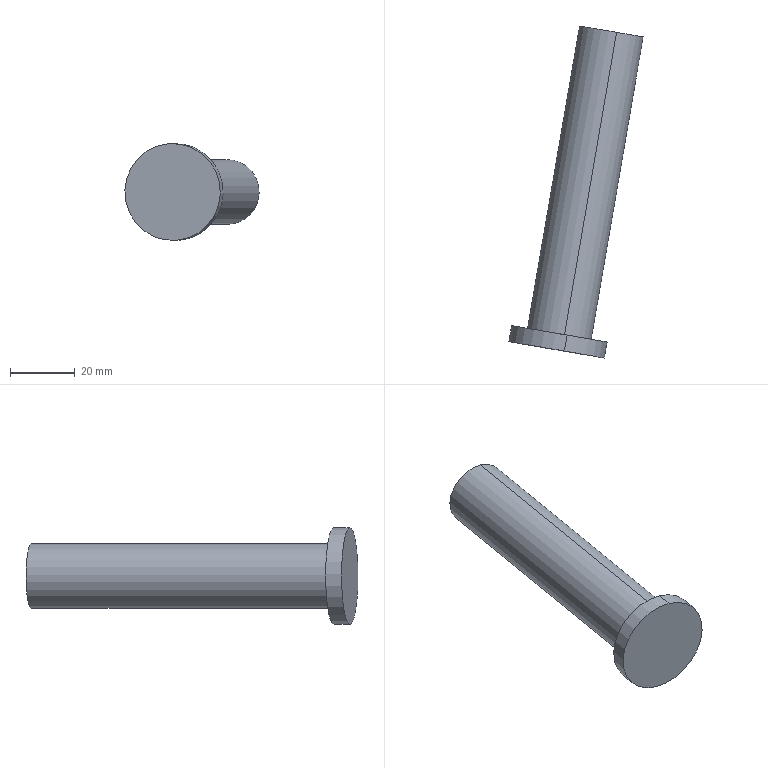Component | SolidWorks | 7xiao-1 | 1 solid | 7 faces | box 41.59 x 102.79 x 30 mm | volume 33379 mm3 | cylinder 4 | plane 3 | commonest cylinder face diameters 30 x2 20 x2 | material 45
build123d program:
from build123d import *

# Parameters (mm, degrees)
SKETCH1_3_R         = 10
BOSS_EXTRUDE1_DEPTH = 100
SKETCH1_3_2_R       = 15
SKETCH1_3_2_R_2     = 10
BOSS_EXTRUDE2_DEPTH = 5


with BuildPart() as part:
    # Sketch1_3 → Boss-Extrude1 (new body)
    with BuildSketch(Plane.XY):
        Circle(SKETCH1_3_R)
    extrude(amount=BOSS_EXTRUDE1_DEPTH)

    # Sketch1_3 2 → Boss-Extrude2 (add)
    with BuildSketch(Plane.XY):
        Circle(SKETCH1_3_2_R)
        Circle(SKETCH1_3_2_R_2, mode=Mode.SUBTRACT)
    extrude(amount=BOSS_EXTRUDE2_DEPTH)


solid = part.part

# Placed as in the assembly
solid = solid.moved(Location((136.99, -853.32, 617.679), (-90, 9.76, -94.621)))
STEP:
#1=COLOUR_RGB('',0.7922,0.8196,0.9333);
#2=FILL_AREA_STYLE_COLOUR('',#1);
#3=FILL_AREA_STYLE('',(#2));
#4=SURFACE_STYLE_FILL_AREA(#3);
#5=SURFACE_SIDE_STYLE('',(#4));
#6=SURFACE_STYLE_USAGE(.BOTH.,#5);
#7=PRESENTATION_STYLE_ASSIGNMENT((#6));
#8=CARTESIAN_POINT('',(5.332,-33.385,23.735));
#9=VERTEX_POINT('',#8);
#10=CARTESIAN_POINT('',(5.522,-33.418,24.901));
#11=VERTEX_POINT('',#10);
#12=CARTESIAN_POINT('',(5.427,-33.401,24.318));
#13=DIRECTION('',(0.1695,0.9855,0.));
#14=DIRECTION('',(-0.1609,0.02767,-0.9866));
#15=AXIS2_PLACEMENT_3D('',#12,#13,#14);
#16=CIRCLE('',#15,0.5906);
#17=EDGE_CURVE('',#9,#11,#16,.T.);
#18=ORIENTED_EDGE('',*,*,#17,.F.);
#19=CARTESIAN_POINT('',(5.298,-33.579,23.735));
#20=VERTEX_POINT('',#19);
#21=CARTESIAN_POINT('',(5.332,-33.385,23.735));
#22=DIRECTION('',(-0.1695,-0.9855,-0.));
#23=VECTOR('',#22,39.37);
#24=LINE('',#21,#23);
#25=EDGE_CURVE('',#9,#20,#24,.T.);
#26=ORIENTED_EDGE('',*,*,#25,.T.);
#27=CARTESIAN_POINT('',(5.488,-33.612,24.901));
#28=VERTEX_POINT('',#27);
#29=CARTESIAN_POINT('',(5.393,-33.595,24.318));
#30=DIRECTION('',(0.1695,0.9855,0.));
#31=DIRECTION('',(-0.1609,0.02767,-0.9866));
#32=AXIS2_PLACEMENT_3D('',#29,#30,#31);
#33=CIRCLE('',#32,0.5906);
#34=EDGE_CURVE('',#20,#28,#33,.T.);
#35=ORIENTED_EDGE('',*,*,#34,.T.);
#36=CARTESIAN_POINT('',(5.522,-33.418,24.901));
#37=DIRECTION('',(-0.1695,-0.9855,-0.));
#38=VECTOR('',#37,39.37);
#39=LINE('',#36,#38);
#40=EDGE_CURVE('',#11,#28,#39,.T.);
#41=ORIENTED_EDGE('',*,*,#40,.F.);
#42=EDGE_LOOP('',(#18,#26,#35,#41));
#43=FACE_OUTER_BOUND('',#42,.T.);
#44=CARTESIAN_POINT('',(5.427,-33.401,24.318));
#45=DIRECTION('',(-0.1695,-0.9855,-0.));
#46=DIRECTION('',(0.1609,-0.02767,0.9866));
#47=AXIS2_PLACEMENT_3D('',#44,#45,#46);
#48=CYLINDRICAL_SURFACE('',#47,0.5906);
#49=ADVANCED_FACE('',(#43),#48,.T.);
#50=CARTESIAN_POINT('',(5.997,-29.704,23.93));
#51=VERTEX_POINT('',#50);
#52=CARTESIAN_POINT('',(6.124,-29.726,24.707));
#53=VERTEX_POINT('',#52);
#54=CARTESIAN_POINT('',(6.061,-29.715,24.318));
#55=DIRECTION('',(0.1695,0.9855,0.));
#56=DIRECTION('',(-0.1609,0.02767,-0.9866));
#57=AXIS2_PLACEMENT_3D('',#54,#55,#56);
#58=CIRCLE('',#57,0.3937);
#59=EDGE_CURVE('',#51,#53,#58,.T.);
#60=ORIENTED_EDGE('',*,*,#59,.F.);
#61=CARTESIAN_POINT('',(5.363,-33.39,23.93));
#62=VERTEX_POINT('',#61);
#63=CARTESIAN_POINT('',(5.997,-29.704,23.93));
#64=DIRECTION('',(-0.1695,-0.9855,-0.));
#65=VECTOR('',#64,39.37);
#66=LINE('',#63,#65);
#67=EDGE_CURVE('',#51,#62,#66,.T.);
#68=ORIENTED_EDGE('',*,*,#67,.T.);
#69=CARTESIAN_POINT('',(5.49,-33.412,24.707));
#70=VERTEX_POINT('',#69);
#71=CARTESIAN_POINT('',(5.427,-33.401,24.318));
#72=DIRECTION('',(0.1695,0.9855,0.));
#73=DIRECTION('',(-0.1609,0.02767,-0.9866));
#74=AXIS2_PLACEMENT_3D('',#71,#72,#73);
#75=CIRCLE('',#74,0.3937);
#76=EDGE_CURVE('',#62,#70,#75,.T.);
#77=ORIENTED_EDGE('',*,*,#76,.T.);
#78=CARTESIAN_POINT('',(6.124,-29.726,24.707));
#79=DIRECTION('',(-0.1695,-0.9855,-0.));
#80=VECTOR('',#79,39.37);
#81=LINE('',#78,#80);
#82=EDGE_CURVE('',#53,#70,#81,.T.);
#83=ORIENTED_EDGE('',*,*,#82,.F.);
#84=EDGE_LOOP('',(#60,#68,#77,#83));
#85=FACE_OUTER_BOUND('',#84,.T.);
#86=CARTESIAN_POINT('',(6.061,-29.715,24.318));
#87=DIRECTION('',(-0.1695,-0.9855,-0.));
#88=DIRECTION('',(0.1609,-0.02767,0.9866));
#89=AXIS2_PLACEMENT_3D('',#86,#87,#88);
#90=CYLINDRICAL_SURFACE('',#89,0.3937);
#91=ADVANCED_FACE('',(#85),#90,.T.);
#92=ORIENTED_EDGE('',*,*,#67,.F.);
#93=CARTESIAN_POINT('',(6.061,-29.715,24.318));
#94=DIRECTION('',(0.1695,0.9855,0.));
#95=DIRECTION('',(-0.1609,0.02767,-0.9866));
#96=AXIS2_PLACEMENT_3D('',#93,#94,#95);
#97=CIRCLE('',#96,0.3937);
#98=EDGE_CURVE('',#53,#51,#97,.T.);
#99=ORIENTED_EDGE('',*,*,#98,.F.);
#100=ORIENTED_EDGE('',*,*,#82,.T.);
#101=CARTESIAN_POINT('',(5.427,-33.401,24.318));
#102=DIRECTION('',(0.1695,0.9855,0.));
#103=DIRECTION('',(-0.1609,0.02767,-0.9866));
#104=AXIS2_PLACEMENT_3D('',#101,#102,#103);
#105=CIRCLE('',#104,0.3937);
#106=EDGE_CURVE('',#70,#62,#105,.T.);
#107=ORIENTED_EDGE('',*,*,#106,.T.);
#108=EDGE_LOOP('',(#92,#99,#100,#107));
#109=FACE_OUTER_BOUND('',#108,.T.);
#110=CARTESIAN_POINT('',(6.061,-29.715,24.318));
#111=DIRECTION('',(-0.1695,-0.9855,-0.));
#112=DIRECTION('',(0.1609,-0.02767,0.9866));
#113=AXIS2_PLACEMENT_3D('',#110,#111,#112);
#114=CYLINDRICAL_SURFACE('',#113,0.3937);
#115=ADVANCED_FACE('',(#109),#114,.T.);
#116=ORIENTED_EDGE('',*,*,#98,.T.);
#117=ORIENTED_EDGE('',*,*,#59,.T.);
#118=EDGE_LOOP('',(#116,#117));
#119=FACE_OUTER_BOUND('',#118,.T.);
#120=CARTESIAN_POINT('',(6.061,-29.715,24.318));
#121=DIRECTION('',(0.1695,0.9855,0.));
#122=DIRECTION('',(-0.1609,0.02767,-0.9866));
#123=AXIS2_PLACEMENT_3D('',#120,#121,#122);
#124=PLANE('',#123);
#125=ADVANCED_FACE('',(#119),#124,.T.);
#126=CARTESIAN_POINT('',(5.427,-33.401,24.318));
#127=DIRECTION('',(0.1695,0.9855,0.));
#128=DIRECTION('',(-0.1609,0.02767,-0.9866));
#129=AXIS2_PLACEMENT_3D('',#126,#127,#128);
#130=CIRCLE('',#129,0.5906);
#131=EDGE_CURVE('',#11,#9,#130,.T.);
#132=ORIENTED_EDGE('',*,*,#131,.T.);
#133=ORIENTED_EDGE('',*,*,#17,.T.);
#134=EDGE_LOOP('',(#132,#133));
#135=FACE_OUTER_BOUND('',#134,.T.);
#136=ORIENTED_EDGE('',*,*,#106,.F.);
#137=ORIENTED_EDGE('',*,*,#76,.F.);
#138=EDGE_LOOP('',(#136,#137));
#139=FACE_BOUND('',#138,.T.);
#140=CARTESIAN_POINT('',(5.427,-33.401,24.318));
#141=DIRECTION('',(0.1695,0.9855,0.));
#142=DIRECTION('',(-0.1609,0.02767,-0.9866));
#143=AXIS2_PLACEMENT_3D('',#140,#141,#142);
#144=PLANE('',#143);
#145=ADVANCED_FACE('',(#135,#139),#144,.T.);
#146=ORIENTED_EDGE('',*,*,#25,.F.);
#147=ORIENTED_EDGE('',*,*,#131,.F.);
#148=ORIENTED_EDGE('',*,*,#40,.T.);
#149=CARTESIAN_POINT('',(5.393,-33.595,24.318));
#150=DIRECTION('',(0.1695,0.9855,0.));
#151=DIRECTION('',(-0.1609,0.02767,-0.9866));
#152=AXIS2_PLACEMENT_3D('',#149,#150,#151);
#153=CIRCLE('',#152,0.5906);
#154=EDGE_CURVE('',#28,#20,#153,.T.);
#155=ORIENTED_EDGE('',*,*,#154,.T.);
#156=EDGE_LOOP('',(#146,#147,#148,#155));
#157=FACE_OUTER_BOUND('',#156,.T.);
#158=CARTESIAN_POINT('',(5.427,-33.401,24.318));
#159=DIRECTION('',(-0.1695,-0.9855,-0.));
#160=DIRECTION('',(0.1609,-0.02767,0.9866));
#161=AXIS2_PLACEMENT_3D('',#158,#159,#160);
#162=CYLINDRICAL_SURFACE('',#161,0.5906);
#163=ADVANCED_FACE('',(#157),#162,.T.);
#164=ORIENTED_EDGE('',*,*,#154,.F.);
#165=ORIENTED_EDGE('',*,*,#34,.F.);
#166=EDGE_LOOP('',(#164,#165));
#167=FACE_OUTER_BOUND('',#166,.T.);
#168=CARTESIAN_POINT('',(5.393,-33.595,24.318));
#169=DIRECTION('',(0.1695,0.9855,0.));
#170=DIRECTION('',(-0.1609,0.02767,-0.9866));
#171=AXIS2_PLACEMENT_3D('',#168,#169,#170);
#172=PLANE('',#171);
#173=ADVANCED_FACE('',(#167),#172,.F.);
#174=CLOSED_SHELL('',(#49,#91,#115,#125,#145,#163,#173));
#175=MANIFOLD_SOLID_BREP('',#174);
#176=STYLED_ITEM('',(#7),#175);
#177=PRESENTATION_LAYER_ASSIGNMENT('','',(#176));
#178=CARTESIAN_POINT('',(0.,0.,0.));
#179=DIRECTION('',(0.,0.,1.));
#180=DIRECTION('',(1.,0.,0.));
#181=AXIS2_PLACEMENT_3D('',#178,#179,#180);
#182=(LENGTH_UNIT()NAMED_UNIT(*)SI_UNIT($,.METRE.));
#183=LENGTH_MEASURE_WITH_UNIT(LENGTH_MEASURE(0.0254),#182);
#184=DIMENSIONAL_EXPONENTS(1.,0.,0.,0.,0.,0.,0.);
#185=(CONVERSION_BASED_UNIT('',#183)LENGTH_UNIT()NAMED_UNIT(#184));
#186=UNCERTAINTY_MEASURE_WITH_UNIT(LENGTH_MEASURE(0.00001),#185,'','');
#187=(NAMED_UNIT(*)PLANE_ANGLE_UNIT()SI_UNIT($,.RADIAN.));
#188=(NAMED_UNIT(*)SI_UNIT($,.STERADIAN.)SOLID_ANGLE_UNIT());
#189=(GEOMETRIC_REPRESENTATION_CONTEXT(3)GLOBAL_UNCERTAINTY_ASSIGNED_CONTEXT((#186))GLOBAL_UNIT_ASSIGNED_CONTEXT((#185,#187,#188))REPRESENTATION_CONTEXT('',''));
#190=ADVANCED_BREP_SHAPE_REPRESENTATION('',(#175,#181),#189);
#191=(LENGTH_UNIT()NAMED_UNIT(*)SI_UNIT($,.METRE.));
#192=LENGTH_MEASURE_WITH_UNIT(LENGTH_MEASURE(0.0254),#191);
#193=DIMENSIONAL_EXPONENTS(1.,0.,0.,0.,0.,0.,0.);
#194=(CONVERSION_BASED_UNIT('',#192)LENGTH_UNIT()NAMED_UNIT(#193));
#195=UNCERTAINTY_MEASURE_WITH_UNIT(LENGTH_MEASURE(0.00001),#194,'','');
#196=(NAMED_UNIT(*)PLANE_ANGLE_UNIT()SI_UNIT($,.RADIAN.));
#197=(NAMED_UNIT(*)SI_UNIT($,.STERADIAN.)SOLID_ANGLE_UNIT());
#198=(GEOMETRIC_REPRESENTATION_CONTEXT(3)GLOBAL_UNCERTAINTY_ASSIGNED_CONTEXT((#195))GLOBAL_UNIT_ASSIGNED_CONTEXT((#194,#196,#197))REPRESENTATION_CONTEXT('',''));
#199=MECHANICAL_DESIGN_GEOMETRIC_PRESENTATION_REPRESENTATION('',(#176),#198);